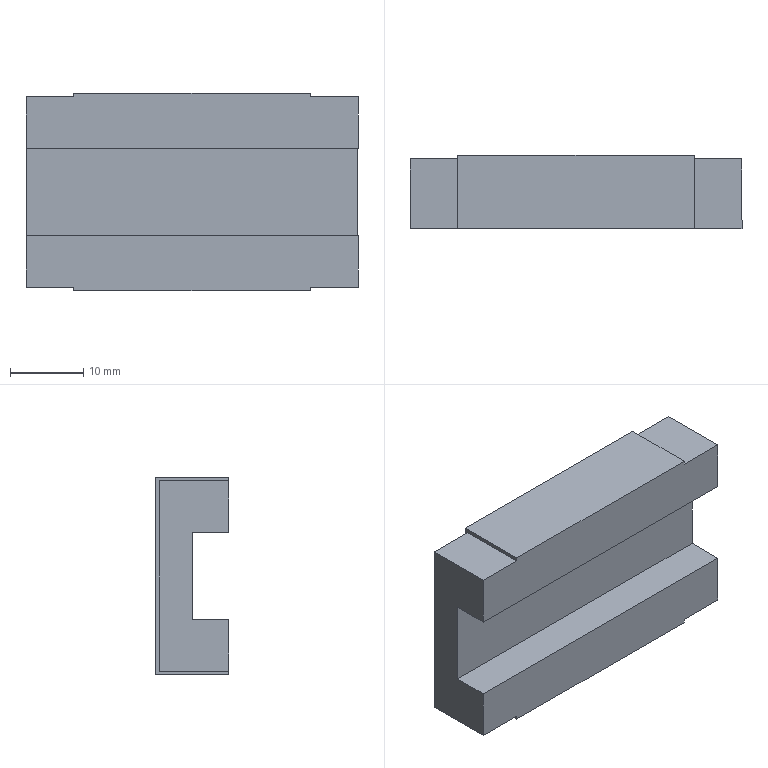Component | SolidWorks | MGN12H1R145Z0C-1_MGN12H-1 | 1 solid | 30 faces | box 45.4 x 10 x 27 mm | volume 9169 mm3 | plane 22 | cylinder 8 | commonest cylinder face diameters 2.3 x8 | material Plain Carbon Steel
build123d program:
from build123d import *

# Parameters (mm, degrees)
SKETCH1_W               = 27
SKETCH1_H               = 10
EXTRUDE1_DEPTH          = 22.7
SKETCH2_W               = 12
SKETCH2_H               = 5
CUT_EXTRUDE1_DEPTH      = 49.409
SKETCH3_W               = 27
SKETCH3_H               = 6.5
CUT_EXTRUDE2_DEPTH      = 0.5
SKETCH4_W               = 0.5
SKETCH4_H               = 6.5
CUT_EXTRUDE3_DEPTH      = 29.068
MIRROR2_COPY_1_SKETCH_W = 0.5
MIRROR2_COPY_1_SKETCH_H = 6.5
MIRROR2_COPY_1_DEPTH    = 29.068
SKETCH5_R               = 1.15
CUT_EXTRUDE4_DEPTH      = 4
LPATTERN1_COUNT         = 2
LPATTERN1_PITCH         = 20
LPATTERN1_COUNT_DIR2    = 2
LPATTERN1_PITCH_DIR2    = 20


with BuildPart() as part:
    # Sketch1 → Extrude1 (new, symmetric)
    with BuildSketch(Plane.XY):
        with Locations((0, 5)):
            Rectangle(SKETCH1_W, SKETCH1_H)
    extrude(amount=EXTRUDE1_DEPTH, both=True)

    # Sketch2 → Cut-Extrude1 (cut, through all)
    with BuildSketch(Plane.XY.offset(22.7)):
        with Locations((0, 2.5)):
            Rectangle(SKETCH2_W, SKETCH2_H)
    extrude(amount=-CUT_EXTRUDE1_DEPTH, mode=Mode.SUBTRACT)

    # Sketch3 → Cut-Extrude2 (cut)
    with BuildSketch(Plane(origin=(0, 10, 0), x_dir=(-1, 0, 0), z_dir=(0, 1, 0))):
        with Locations((0, 19.45)):
            Rectangle(SKETCH3_W, SKETCH3_H)
    cut_extrude2 = extrude(amount=-CUT_EXTRUDE2_DEPTH, mode=Mode.SUBTRACT)

    # Sketch4 → Cut-Extrude3 (cut, through all)
    with BuildSketch(Plane(origin=(0, 9.5, 0), x_dir=(-1, 0, 0), z_dir=(0, 1, 0))):
        with Locations((13.25, 19.45)):
            Rectangle(SKETCH4_W, SKETCH4_H)
    cut_extrude3 = extrude(amount=-CUT_EXTRUDE3_DEPTH, mode=Mode.SUBTRACT)

    # Mirror1: Cut-Extrude3 across plane
    add(cut_extrude3.mirror(Plane(origin=(0, 0, 0), x_dir=(0, 0, 1), z_dir=(1, 0, 0))), mode=Mode.SUBTRACT)

    # Mirror2: Cut-Extrude2, Cut-Extrude3 across plane
    add(cut_extrude2.mirror(Plane.XY), mode=Mode.SUBTRACT)
    add(cut_extrude3.mirror(Plane.XY), mode=Mode.SUBTRACT)

    # Mirror2 copy 1 sketch → Mirror2 copy 1 (cut, through all)
    with BuildSketch(Plane(origin=(0, 9.5, 0), x_dir=(1, 0, 0), z_dir=(0, 1, 0))):
        with Locations((13.25, 19.45)):
            Rectangle(MIRROR2_COPY_1_SKETCH_W, MIRROR2_COPY_1_SKETCH_H)
    extrude(amount=-MIRROR2_COPY_1_DEPTH, mode=Mode.SUBTRACT)

    # Sketch5 → Cut-Extrude4 (cut)
    with BuildSketch(Plane(origin=(0, 10, 0), x_dir=(-1, 0, 0), z_dir=(0, 1, 0))):
        with Locations(Location((-10, 10, 0), (0, 0, 90))):
            Circle(SKETCH5_R)
    cut_extrude4 = extrude(amount=-CUT_EXTRUDE4_DEPTH, mode=Mode.SUBTRACT)

    # LPattern1: Cut-Extrude4 2 × 2
    with Locations(*[(-i * LPATTERN1_PITCH, 0, -j * LPATTERN1_PITCH_DIR2) for i in range(LPATTERN1_COUNT) for j in range(LPATTERN1_COUNT_DIR2) if (i, j) != (0, 0)]):
        add(cut_extrude4, mode=Mode.SUBTRACT)


solid = part.part

# Placed as in the assembly
solid = solid.moved(Location((104.77, 11.768, 38.329), (0, 90, 0)))
STEP:
#1=COLOUR_RGB('',0.7922,0.8196,0.9333);
#2=FILL_AREA_STYLE_COLOUR('',#1);
#3=FILL_AREA_STYLE('',(#2));
#4=SURFACE_STYLE_FILL_AREA(#3);
#5=SURFACE_SIDE_STYLE('',(#4));
#6=SURFACE_STYLE_USAGE(.BOTH.,#5);
#7=PRESENTATION_STYLE_ASSIGNMENT((#6));
#8=CARTESIAN_POINT('',(4.564,0.6995,1.115));
#9=VERTEX_POINT('',#8);
#10=CARTESIAN_POINT('',(4.473,0.6995,1.115));
#11=VERTEX_POINT('',#10);
#12=CARTESIAN_POINT('',(4.519,0.6995,1.115));
#13=DIRECTION('',(-0.,1.,-0.));
#14=DIRECTION('',(-1.,0.,0.));
#15=AXIS2_PLACEMENT_3D('',#12,#13,#14);
#16=CIRCLE('',#15,0.04528);
#17=EDGE_CURVE('',#9,#11,#16,.T.);
#18=ORIENTED_EDGE('',*,*,#17,.F.);
#19=CARTESIAN_POINT('',(4.564,0.857,1.115));
#20=VERTEX_POINT('',#19);
#21=CARTESIAN_POINT('',(4.564,0.6995,1.115));
#22=DIRECTION('',(-0.,1.,-0.));
#23=VECTOR('',#22,39.37);
#24=LINE('',#21,#23);
#25=EDGE_CURVE('',#9,#20,#24,.T.);
#26=ORIENTED_EDGE('',*,*,#25,.T.);
#27=CARTESIAN_POINT('',(4.473,0.857,1.115));
#28=VERTEX_POINT('',#27);
#29=CARTESIAN_POINT('',(4.519,0.857,1.115));
#30=DIRECTION('',(-0.,1.,-0.));
#31=DIRECTION('',(-1.,0.,0.));
#32=AXIS2_PLACEMENT_3D('',#29,#30,#31);
#33=CIRCLE('',#32,0.04528);
#34=EDGE_CURVE('',#20,#28,#33,.T.);
#35=ORIENTED_EDGE('',*,*,#34,.T.);
#36=CARTESIAN_POINT('',(4.473,0.6995,1.115));
#37=DIRECTION('',(-0.,1.,-0.));
#38=VECTOR('',#37,39.37);
#39=LINE('',#36,#38);
#40=EDGE_CURVE('',#11,#28,#39,.T.);
#41=ORIENTED_EDGE('',*,*,#40,.F.);
#42=EDGE_LOOP('',(#18,#26,#35,#41));
#43=FACE_OUTER_BOUND('',#42,.T.);
#44=CARTESIAN_POINT('',(4.519,0.6995,1.115));
#45=DIRECTION('',(-0.,1.,-0.));
#46=DIRECTION('',(-1.,0.,0.));
#47=AXIS2_PLACEMENT_3D('',#44,#45,#46);
#48=CYLINDRICAL_SURFACE('',#47,0.04528);
#49=ADVANCED_FACE('',(#43),#48,.F.);
#50=CARTESIAN_POINT('',(4.564,0.6995,1.903));
#51=VERTEX_POINT('',#50);
#52=CARTESIAN_POINT('',(4.473,0.6995,1.903));
#53=VERTEX_POINT('',#52);
#54=CARTESIAN_POINT('',(4.519,0.6995,1.903));
#55=DIRECTION('',(-0.,1.,-0.));
#56=DIRECTION('',(-1.,0.,0.));
#57=AXIS2_PLACEMENT_3D('',#54,#55,#56);
#58=CIRCLE('',#57,0.04528);
#59=EDGE_CURVE('',#51,#53,#58,.T.);
#60=ORIENTED_EDGE('',*,*,#59,.F.);
#61=CARTESIAN_POINT('',(4.564,0.857,1.903));
#62=VERTEX_POINT('',#61);
#63=CARTESIAN_POINT('',(4.564,0.6995,1.903));
#64=DIRECTION('',(-0.,1.,-0.));
#65=VECTOR('',#64,39.37);
#66=LINE('',#63,#65);
#67=EDGE_CURVE('',#51,#62,#66,.T.);
#68=ORIENTED_EDGE('',*,*,#67,.T.);
#69=CARTESIAN_POINT('',(4.473,0.857,1.903));
#70=VERTEX_POINT('',#69);
#71=CARTESIAN_POINT('',(4.519,0.857,1.903));
#72=DIRECTION('',(-0.,1.,-0.));
#73=DIRECTION('',(-1.,0.,0.));
#74=AXIS2_PLACEMENT_3D('',#71,#72,#73);
#75=CIRCLE('',#74,0.04528);
#76=EDGE_CURVE('',#62,#70,#75,.T.);
#77=ORIENTED_EDGE('',*,*,#76,.T.);
#78=CARTESIAN_POINT('',(4.473,0.6995,1.903));
#79=DIRECTION('',(-0.,1.,-0.));
#80=VECTOR('',#79,39.37);
#81=LINE('',#78,#80);
#82=EDGE_CURVE('',#53,#70,#81,.T.);
#83=ORIENTED_EDGE('',*,*,#82,.F.);
#84=EDGE_LOOP('',(#60,#68,#77,#83));
#85=FACE_OUTER_BOUND('',#84,.T.);
#86=CARTESIAN_POINT('',(4.519,0.6995,1.903));
#87=DIRECTION('',(-0.,1.,-0.));
#88=DIRECTION('',(-1.,0.,0.));
#89=AXIS2_PLACEMENT_3D('',#86,#87,#88);
#90=CYLINDRICAL_SURFACE('',#89,0.04528);
#91=ADVANCED_FACE('',(#85),#90,.F.);
#92=CARTESIAN_POINT('',(3.776,0.6995,1.115));
#93=VERTEX_POINT('',#92);
#94=CARTESIAN_POINT('',(3.686,0.6995,1.115));
#95=VERTEX_POINT('',#94);
#96=CARTESIAN_POINT('',(3.731,0.6995,1.115));
#97=DIRECTION('',(-0.,1.,-0.));
#98=DIRECTION('',(-1.,0.,0.));
#99=AXIS2_PLACEMENT_3D('',#96,#97,#98);
#100=CIRCLE('',#99,0.04528);
#101=EDGE_CURVE('',#93,#95,#100,.T.);
#102=ORIENTED_EDGE('',*,*,#101,.F.);
#103=CARTESIAN_POINT('',(3.776,0.857,1.115));
#104=VERTEX_POINT('',#103);
#105=CARTESIAN_POINT('',(3.776,0.6995,1.115));
#106=DIRECTION('',(-0.,1.,-0.));
#107=VECTOR('',#106,39.37);
#108=LINE('',#105,#107);
#109=EDGE_CURVE('',#93,#104,#108,.T.);
#110=ORIENTED_EDGE('',*,*,#109,.T.);
#111=CARTESIAN_POINT('',(3.686,0.857,1.115));
#112=VERTEX_POINT('',#111);
#113=CARTESIAN_POINT('',(3.731,0.857,1.115));
#114=DIRECTION('',(-0.,1.,-0.));
#115=DIRECTION('',(-1.,0.,0.));
#116=AXIS2_PLACEMENT_3D('',#113,#114,#115);
#117=CIRCLE('',#116,0.04528);
#118=EDGE_CURVE('',#104,#112,#117,.T.);
#119=ORIENTED_EDGE('',*,*,#118,.T.);
#120=CARTESIAN_POINT('',(3.686,0.6995,1.115));
#121=DIRECTION('',(-0.,1.,-0.));
#122=VECTOR('',#121,39.37);
#123=LINE('',#120,#122);
#124=EDGE_CURVE('',#95,#112,#123,.T.);
#125=ORIENTED_EDGE('',*,*,#124,.F.);
#126=EDGE_LOOP('',(#102,#110,#119,#125));
#127=FACE_OUTER_BOUND('',#126,.T.);
#128=CARTESIAN_POINT('',(3.731,0.6995,1.115));
#129=DIRECTION('',(-0.,1.,-0.));
#130=DIRECTION('',(-1.,0.,0.));
#131=AXIS2_PLACEMENT_3D('',#128,#129,#130);
#132=CYLINDRICAL_SURFACE('',#131,0.04528);
#133=ADVANCED_FACE('',(#127),#132,.F.);
#134=CARTESIAN_POINT('',(3.776,0.6995,1.903));
#135=VERTEX_POINT('',#134);
#136=CARTESIAN_POINT('',(3.686,0.6995,1.903));
#137=VERTEX_POINT('',#136);
#138=CARTESIAN_POINT('',(3.731,0.6995,1.903));
#139=DIRECTION('',(-0.,1.,-0.));
#140=DIRECTION('',(-1.,0.,0.));
#141=AXIS2_PLACEMENT_3D('',#138,#139,#140);
#142=CIRCLE('',#141,0.04528);
#143=EDGE_CURVE('',#135,#137,#142,.T.);
#144=ORIENTED_EDGE('',*,*,#143,.F.);
#145=CARTESIAN_POINT('',(3.776,0.857,1.903));
#146=VERTEX_POINT('',#145);
#147=CARTESIAN_POINT('',(3.776,0.6995,1.903));
#148=DIRECTION('',(-0.,1.,-0.));
#149=VECTOR('',#148,39.37);
#150=LINE('',#147,#149);
#151=EDGE_CURVE('',#135,#146,#150,.T.);
#152=ORIENTED_EDGE('',*,*,#151,.T.);
#153=CARTESIAN_POINT('',(3.686,0.857,1.903));
#154=VERTEX_POINT('',#153);
#155=CARTESIAN_POINT('',(3.731,0.857,1.903));
#156=DIRECTION('',(-0.,1.,-0.));
#157=DIRECTION('',(-1.,0.,0.));
#158=AXIS2_PLACEMENT_3D('',#155,#156,#157);
#159=CIRCLE('',#158,0.04528);
#160=EDGE_CURVE('',#146,#154,#159,.T.);
#161=ORIENTED_EDGE('',*,*,#160,.T.);
#162=CARTESIAN_POINT('',(3.686,0.6995,1.903));
#163=DIRECTION('',(-0.,1.,-0.));
#164=VECTOR('',#163,39.37);
#165=LINE('',#162,#164);
#166=EDGE_CURVE('',#137,#154,#165,.T.);
#167=ORIENTED_EDGE('',*,*,#166,.F.);
#168=EDGE_LOOP('',(#144,#152,#161,#167));
#169=FACE_OUTER_BOUND('',#168,.T.);
#170=CARTESIAN_POINT('',(3.731,0.6995,1.903));
#171=DIRECTION('',(-0.,1.,-0.));
#172=DIRECTION('',(-1.,0.,0.));
#173=AXIS2_PLACEMENT_3D('',#170,#171,#172);
#174=CYLINDRICAL_SURFACE('',#173,0.04528);
#175=ADVANCED_FACE('',(#169),#174,.F.);
#176=CARTESIAN_POINT('',(4.763,0.4633,0.9775));
#177=VERTEX_POINT('',#176);
#178=CARTESIAN_POINT('',(4.763,0.857,0.9775));
#179=VERTEX_POINT('',#178);
#180=CARTESIAN_POINT('',(4.763,0.8373,0.9775));
#181=DIRECTION('',(-0.,1.,-0.));
#182=VECTOR('',#181,39.37);
#183=LINE('',#180,#182);
#184=EDGE_CURVE('',#177,#179,#183,.T.);
#185=ORIENTED_EDGE('',*,*,#184,.F.);
#186=CARTESIAN_POINT('',(3.487,0.4633,0.9775));
#187=VERTEX_POINT('',#186);
#188=CARTESIAN_POINT('',(3.231,0.4633,0.9775));
#189=DIRECTION('',(1.,0.,-0.));
#190=VECTOR('',#189,39.37);
#191=LINE('',#188,#190);
#192=EDGE_CURVE('',#187,#177,#191,.T.);
#193=ORIENTED_EDGE('',*,*,#192,.F.);
#194=CARTESIAN_POINT('',(3.487,0.857,0.9775));
#195=VERTEX_POINT('',#194);
#196=CARTESIAN_POINT('',(3.487,0.8373,0.9775));
#197=DIRECTION('',(-0.,1.,-0.));
#198=VECTOR('',#197,39.37);
#199=LINE('',#196,#198);
#200=EDGE_CURVE('',#187,#195,#199,.T.);
#201=ORIENTED_EDGE('',*,*,#200,.T.);
#202=CARTESIAN_POINT('',(3.231,0.857,0.9775));
#203=DIRECTION('',(1.,0.,-0.));
#204=VECTOR('',#203,39.37);
#205=LINE('',#202,#204);
#206=EDGE_CURVE('',#195,#179,#205,.T.);
#207=ORIENTED_EDGE('',*,*,#206,.T.);
#208=EDGE_LOOP('',(#185,#193,#201,#207));
#209=FACE_OUTER_BOUND('',#208,.T.);
#210=CARTESIAN_POINT('',(3.231,0.857,0.9775));
#211=DIRECTION('',(0.,0.,1.));
#212=DIRECTION('',(-0.,1.,-0.));
#213=AXIS2_PLACEMENT_3D('',#210,#211,#212);
#214=PLANE('',#213);
#215=ADVANCED_FACE('',(#209),#214,.F.);
#216=CARTESIAN_POINT('',(5.019,0.4633,0.9972));
#217=VERTEX_POINT('',#216);
#218=CARTESIAN_POINT('',(5.019,0.8373,0.9972));
#219=VERTEX_POINT('',#218);
#220=CARTESIAN_POINT('',(5.019,0.4633,0.9972));
#221=DIRECTION('',(-0.,1.,-0.));
#222=VECTOR('',#221,39.37);
#223=LINE('',#220,#222);
#224=EDGE_CURVE('',#217,#219,#223,.T.);
#225=ORIENTED_EDGE('',*,*,#224,.T.);
#226=CARTESIAN_POINT('',(5.019,0.8373,2.021));
#227=VERTEX_POINT('',#226);
#228=CARTESIAN_POINT('',(5.019,0.8373,2.041));
#229=DIRECTION('',(0.,0.,1.));
#230=VECTOR('',#229,39.37);
#231=LINE('',#228,#230);
#232=EDGE_CURVE('',#219,#227,#231,.T.);
#233=ORIENTED_EDGE('',*,*,#232,.T.);
#234=CARTESIAN_POINT('',(5.019,0.4633,2.021));
#235=VERTEX_POINT('',#234);
#236=CARTESIAN_POINT('',(5.019,0.4633,2.021));
#237=DIRECTION('',(-0.,1.,-0.));
#238=VECTOR('',#237,39.37);
#239=LINE('',#236,#238);
#240=EDGE_CURVE('',#235,#227,#239,.T.);
#241=ORIENTED_EDGE('',*,*,#240,.F.);
#242=CARTESIAN_POINT('',(5.019,0.4633,1.745));
#243=VERTEX_POINT('',#242);
#244=CARTESIAN_POINT('',(5.019,0.4633,0.9775));
#245=DIRECTION('',(0.,0.,1.));
#246=VECTOR('',#245,39.37);
#247=LINE('',#244,#246);
#248=EDGE_CURVE('',#243,#235,#247,.T.);
#249=ORIENTED_EDGE('',*,*,#248,.F.);
#250=CARTESIAN_POINT('',(5.019,0.6602,1.745));
#251=VERTEX_POINT('',#250);
#252=CARTESIAN_POINT('',(5.019,0.6602,1.745));
#253=DIRECTION('',(-0.,1.,-0.));
#254=VECTOR('',#253,39.37);
#255=LINE('',#252,#254);
#256=EDGE_CURVE('',#243,#251,#255,.T.);
#257=ORIENTED_EDGE('',*,*,#256,.T.);
#258=CARTESIAN_POINT('',(5.019,0.6602,1.273));
#259=VERTEX_POINT('',#258);
#260=CARTESIAN_POINT('',(5.019,0.6602,1.273));
#261=DIRECTION('',(-0.,-0.,-1.));
#262=VECTOR('',#261,39.37);
#263=LINE('',#260,#262);
#264=EDGE_CURVE('',#251,#259,#263,.T.);
#265=ORIENTED_EDGE('',*,*,#264,.T.);
#266=CARTESIAN_POINT('',(5.019,0.4633,1.273));
#267=VERTEX_POINT('',#266);
#268=CARTESIAN_POINT('',(5.019,0.6602,1.273));
#269=DIRECTION('',(0.,-1.,0.));
#270=VECTOR('',#269,39.37);
#271=LINE('',#268,#270);
#272=EDGE_CURVE('',#259,#267,#271,.T.);
#273=ORIENTED_EDGE('',*,*,#272,.T.);
#274=CARTESIAN_POINT('',(5.019,0.4633,0.9775));
#275=DIRECTION('',(0.,0.,1.));
#276=VECTOR('',#275,39.37);
#277=LINE('',#274,#276);
#278=EDGE_CURVE('',#217,#267,#277,.T.);
#279=ORIENTED_EDGE('',*,*,#278,.F.);
#280=EDGE_LOOP('',(#225,#233,#241,#249,#257,#265,#273,#279));
#281=FACE_OUTER_BOUND('',#280,.T.);
#282=CARTESIAN_POINT('',(5.019,0.4633,0.9775));
#283=DIRECTION('',(-1.,-0.,0.));
#284=DIRECTION('',(0.,0.,1.));
#285=AXIS2_PLACEMENT_3D('',#282,#283,#284);
#286=PLANE('',#285);
#287=ADVANCED_FACE('',(#281),#286,.F.);
#288=CARTESIAN_POINT('',(4.763,0.4633,0.9972));
#289=VERTEX_POINT('',#288);
#290=CARTESIAN_POINT('',(5.019,0.4633,0.9972));
#291=DIRECTION('',(-1.,-0.,0.));
#292=VECTOR('',#291,39.37);
#293=LINE('',#290,#292);
#294=EDGE_CURVE('',#217,#289,#293,.T.);
#295=ORIENTED_EDGE('',*,*,#294,.F.);
#296=ORIENTED_EDGE('',*,*,#278,.T.);
#297=CARTESIAN_POINT('',(3.231,0.4633,1.273));
#298=VERTEX_POINT('',#297);
#299=CARTESIAN_POINT('',(5.019,0.4633,1.273));
#300=DIRECTION('',(-1.,-0.,0.));
#301=VECTOR('',#300,39.37);
#302=LINE('',#299,#301);
#303=EDGE_CURVE('',#267,#298,#302,.T.);
#304=ORIENTED_EDGE('',*,*,#303,.T.);
#305=CARTESIAN_POINT('',(3.231,0.4633,0.9972));
#306=VERTEX_POINT('',#305);
#307=CARTESIAN_POINT('',(3.231,0.4633,0.9775));
#308=DIRECTION('',(0.,0.,1.));
#309=VECTOR('',#308,39.37);
#310=LINE('',#307,#309);
#311=EDGE_CURVE('',#306,#298,#310,.T.);
#312=ORIENTED_EDGE('',*,*,#311,.F.);
#313=CARTESIAN_POINT('',(3.487,0.4633,0.9972));
#314=VERTEX_POINT('',#313);
#315=CARTESIAN_POINT('',(3.231,0.4633,0.9972));
#316=DIRECTION('',(1.,0.,-0.));
#317=VECTOR('',#316,39.37);
#318=LINE('',#315,#317);
#319=EDGE_CURVE('',#306,#314,#318,.T.);
#320=ORIENTED_EDGE('',*,*,#319,.T.);
#321=CARTESIAN_POINT('',(3.487,0.4633,0.9775));
#322=DIRECTION('',(-0.,-0.,-1.));
#323=VECTOR('',#322,39.37);
#324=LINE('',#321,#323);
#325=EDGE_CURVE('',#314,#187,#324,.T.);
#326=ORIENTED_EDGE('',*,*,#325,.T.);
#327=ORIENTED_EDGE('',*,*,#192,.T.);
#328=CARTESIAN_POINT('',(4.763,0.4633,0.9775));
#329=DIRECTION('',(-0.,-0.,-1.));
#330=VECTOR('',#329,39.37);
#331=LINE('',#328,#330);
#332=EDGE_CURVE('',#289,#177,#331,.T.);
#333=ORIENTED_EDGE('',*,*,#332,.F.);
#334=EDGE_LOOP('',(#295,#296,#304,#312,#320,#326,#327,#333));
#335=FACE_OUTER_BOUND('',#334,.T.);
#336=CARTESIAN_POINT('',(3.231,0.4633,0.9775));
#337=DIRECTION('',(-0.,1.,-0.));
#338=DIRECTION('',(-1.,-0.,0.));
#339=AXIS2_PLACEMENT_3D('',#336,#337,#338);
#340=PLANE('',#339);
#341=ADVANCED_FACE('',(#335),#340,.F.);
#342=ORIENTED_EDGE('',*,*,#232,.F.);
#343=CARTESIAN_POINT('',(4.763,0.8373,0.9972));
#344=VERTEX_POINT('',#343);
#345=CARTESIAN_POINT('',(5.019,0.8373,0.9972));
#346=DIRECTION('',(-1.,-0.,0.));
#347=VECTOR('',#346,39.37);
#348=LINE('',#345,#347);
#349=EDGE_CURVE('',#219,#344,#348,.T.);
#350=ORIENTED_EDGE('',*,*,#349,.T.);
#351=CARTESIAN_POINT('',(4.763,0.8373,2.021));
#352=VERTEX_POINT('',#351);
#353=CARTESIAN_POINT('',(4.763,0.8373,2.041));
#354=DIRECTION('',(-0.,-0.,-1.));
#355=VECTOR('',#354,39.37);
#356=LINE('',#353,#355);
#357=EDGE_CURVE('',#352,#344,#356,.T.);
#358=ORIENTED_EDGE('',*,*,#357,.F.);
#359=CARTESIAN_POINT('',(5.019,0.8373,2.021));
#360=DIRECTION('',(-1.,-0.,0.));
#361=VECTOR('',#360,39.37);
#362=LINE('',#359,#361);
#363=EDGE_CURVE('',#227,#352,#362,.T.);
#364=ORIENTED_EDGE('',*,*,#363,.F.);
#365=EDGE_LOOP('',(#342,#350,#358,#364));
#366=FACE_OUTER_BOUND('',#365,.T.);
#367=CARTESIAN_POINT('',(4.763,0.8373,2.041));
#368=DIRECTION('',(-0.,1.,-0.));
#369=DIRECTION('',(1.,0.,-0.));
#370=AXIS2_PLACEMENT_3D('',#367,#368,#369);
#371=PLANE('',#370);
#372=ADVANCED_FACE('',(#366),#371,.T.);
#373=CARTESIAN_POINT('',(3.487,0.4633,2.041));
#374=VERTEX_POINT('',#373);
#375=CARTESIAN_POINT('',(4.763,0.4633,2.041));
#376=VERTEX_POINT('',#375);
#377=CARTESIAN_POINT('',(3.231,0.4633,2.041));
#378=DIRECTION('',(1.,0.,-0.));
#379=VECTOR('',#378,39.37);
#380=LINE('',#377,#379);
#381=EDGE_CURVE('',#374,#376,#380,.T.);
#382=ORIENTED_EDGE('',*,*,#381,.T.);
#383=CARTESIAN_POINT('',(4.763,0.857,2.041));
#384=VERTEX_POINT('',#383);
#385=CARTESIAN_POINT('',(4.763,0.8373,2.041));
#386=DIRECTION('',(-0.,1.,-0.));
#387=VECTOR('',#386,39.37);
#388=LINE('',#385,#387);
#389=EDGE_CURVE('',#376,#384,#388,.T.);
#390=ORIENTED_EDGE('',*,*,#389,.T.);
#391=CARTESIAN_POINT('',(3.487,0.857,2.041));
#392=VERTEX_POINT('',#391);
#393=CARTESIAN_POINT('',(3.231,0.857,2.041));
#394=DIRECTION('',(1.,0.,-0.));
#395=VECTOR('',#394,39.37);
#396=LINE('',#393,#395);
#397=EDGE_CURVE('',#392,#384,#396,.T.);
#398=ORIENTED_EDGE('',*,*,#397,.F.);
#399=CARTESIAN_POINT('',(3.487,0.8373,2.041));
#400=DIRECTION('',(-0.,1.,-0.));
#401=VECTOR('',#400,39.37);
#402=LINE('',#399,#401);
#403=EDGE_CURVE('',#374,#392,#402,.T.);
#404=ORIENTED_EDGE('',*,*,#403,.F.);
#405=EDGE_LOOP('',(#382,#390,#398,#404));
#406=FACE_OUTER_BOUND('',#405,.T.);
#407=CARTESIAN_POINT('',(3.231,0.857,2.041));
#408=DIRECTION('',(-0.,-0.,-1.));
#409=DIRECTION('',(0.,-1.,0.));
#410=AXIS2_PLACEMENT_3D('',#407,#408,#409);
#411=PLANE('',#410);
#412=ADVANCED_FACE('',(#406),#411,.F.);
#413=CARTESIAN_POINT('',(3.731,0.857,1.115));
#414=DIRECTION('',(-0.,1.,-0.));
#415=DIRECTION('',(-1.,0.,0.));
#416=AXIS2_PLACEMENT_3D('',#413,#414,#415);
#417=CIRCLE('',#416,0.04528);
#418=EDGE_CURVE('',#112,#104,#417,.T.);
#419=ORIENTED_EDGE('',*,*,#418,.F.);
#420=ORIENTED_EDGE('',*,*,#118,.F.);
#421=EDGE_LOOP('',(#419,#420));
#422=FACE_BOUND('',#421,.T.);
#423=CARTESIAN_POINT('',(3.731,0.857,1.903));
#424=DIRECTION('',(-0.,1.,-0.));
#425=DIRECTION('',(-1.,0.,0.));
#426=AXIS2_PLACEMENT_3D('',#423,#424,#425);
#427=CIRCLE('',#426,0.04528);
#428=EDGE_CURVE('',#154,#146,#427,.T.);
#429=ORIENTED_EDGE('',*,*,#428,.F.);
#430=ORIENTED_EDGE('',*,*,#160,.F.);
#431=EDGE_LOOP('',(#429,#430));
#432=FACE_BOUND('',#431,.T.);
#433=CARTESIAN_POINT('',(4.763,0.857,2.041));
#434=DIRECTION('',(-0.,-0.,-1.));
#435=VECTOR('',#434,39.37);
#436=LINE('',#433,#435);
#437=EDGE_CURVE('',#384,#179,#436,.T.);
#438=ORIENTED_EDGE('',*,*,#437,.T.);
#439=ORIENTED_EDGE('',*,*,#206,.F.);
#440=CARTESIAN_POINT('',(3.487,0.857,2.041));
#441=DIRECTION('',(-0.,-0.,-1.));
#442=VECTOR('',#441,39.37);
#443=LINE('',#440,#442);
#444=EDGE_CURVE('',#392,#195,#443,.T.);
#445=ORIENTED_EDGE('',*,*,#444,.F.);
#446=ORIENTED_EDGE('',*,*,#397,.T.);
#447=EDGE_LOOP('',(#438,#439,#445,#446));
#448=FACE_OUTER_BOUND('',#447,.T.);
#449=CARTESIAN_POINT('',(4.519,0.857,1.903));
#450=DIRECTION('',(-0.,1.,-0.));
#451=DIRECTION('',(-1.,0.,0.));
#452=AXIS2_PLACEMENT_3D('',#449,#450,#451);
#453=CIRCLE('',#452,0.04528);
#454=EDGE_CURVE('',#70,#62,#453,.T.);
#455=ORIENTED_EDGE('',*,*,#454,.F.);
#456=ORIENTED_EDGE('',*,*,#76,.F.);
#457=EDGE_LOOP('',(#455,#456));
#458=FACE_BOUND('',#457,.T.);
#459=CARTESIAN_POINT('',(4.519,0.857,1.115));
#460=DIRECTION('',(-0.,1.,-0.));
#461=DIRECTION('',(-1.,0.,0.));
#462=AXIS2_PLACEMENT_3D('',#459,#460,#461);
#463=CIRCLE('',#462,0.04528);
#464=EDGE_CURVE('',#28,#20,#463,.T.);
#465=ORIENTED_EDGE('',*,*,#464,.F.);
#466=ORIENTED_EDGE('',*,*,#34,.F.);
#467=EDGE_LOOP('',(#465,#466));
#468=FACE_BOUND('',#467,.T.);
#469=CARTESIAN_POINT('',(3.231,0.857,0.9775));
#470=DIRECTION('',(0.,-1.,0.));
#471=DIRECTION('',(1.,0.,-0.));
#472=AXIS2_PLACEMENT_3D('',#469,#470,#471);
#473=PLANE('',#472);
#474=ADVANCED_FACE('',(#422,#432,#448,#458,#468),#473,.F.);
#475=CARTESIAN_POINT('',(3.231,0.4633,1.745));
#476=VERTEX_POINT('',#475);
#477=CARTESIAN_POINT('',(3.231,0.4633,2.021));
#478=VERTEX_POINT('',#477);
#479=CARTESIAN_POINT('',(3.231,0.4633,0.9775));
#480=DIRECTION('',(0.,0.,1.));
#481=VECTOR('',#480,39.37);
#482=LINE('',#479,#481);
#483=EDGE_CURVE('',#476,#478,#482,.T.);
#484=ORIENTED_EDGE('',*,*,#483,.T.);
#485=CARTESIAN_POINT('',(3.231,0.8373,2.021));
#486=VERTEX_POINT('',#485);
#487=CARTESIAN_POINT('',(3.231,0.4633,2.021));
#488=DIRECTION('',(-0.,1.,-0.));
#489=VECTOR('',#488,39.37);
#490=LINE('',#487,#489);
#491=EDGE_CURVE('',#478,#486,#490,.T.);
#492=ORIENTED_EDGE('',*,*,#491,.T.);
#493=CARTESIAN_POINT('',(3.231,0.8373,0.9972));
#494=VERTEX_POINT('',#493);
#495=CARTESIAN_POINT('',(3.231,0.8373,2.041));
#496=DIRECTION('',(0.,0.,1.));
#497=VECTOR('',#496,39.37);
#498=LINE('',#495,#497);
#499=EDGE_CURVE('',#494,#486,#498,.T.);
#500=ORIENTED_EDGE('',*,*,#499,.F.);
#501=CARTESIAN_POINT('',(3.231,0.4633,0.9972));
#502=DIRECTION('',(-0.,1.,-0.));
#503=VECTOR('',#502,39.37);
#504=LINE('',#501,#503);
#505=EDGE_CURVE('',#306,#494,#504,.T.);
#506=ORIENTED_EDGE('',*,*,#505,.F.);
#507=ORIENTED_EDGE('',*,*,#311,.T.);
#508=CARTESIAN_POINT('',(3.231,0.6602,1.273));
#509=VERTEX_POINT('',#508);
#510=CARTESIAN_POINT('',(3.231,0.6602,1.273));
#511=DIRECTION('',(0.,-1.,0.));
#512=VECTOR('',#511,39.37);
#513=LINE('',#510,#512);
#514=EDGE_CURVE('',#509,#298,#513,.T.);
#515=ORIENTED_EDGE('',*,*,#514,.F.);
#516=CARTESIAN_POINT('',(3.231,0.6602,1.745));
#517=VERTEX_POINT('',#516);
#518=CARTESIAN_POINT('',(3.231,0.6602,1.273));
#519=DIRECTION('',(-0.,-0.,-1.));
#520=VECTOR('',#519,39.37);
#521=LINE('',#518,#520);
#522=EDGE_CURVE('',#517,#509,#521,.T.);
#523=ORIENTED_EDGE('',*,*,#522,.F.);
#524=CARTESIAN_POINT('',(3.231,0.6602,1.745));
#525=DIRECTION('',(-0.,1.,-0.));
#526=VECTOR('',#525,39.37);
#527=LINE('',#524,#526);
#528=EDGE_CURVE('',#476,#517,#527,.T.);
#529=ORIENTED_EDGE('',*,*,#528,.F.);
#530=EDGE_LOOP('',(#484,#492,#500,#506,#507,#515,#523,#529));
#531=FACE_OUTER_BOUND('',#530,.T.);
#532=CARTESIAN_POINT('',(3.231,0.4633,0.9775));
#533=DIRECTION('',(-1.,-0.,0.));
#534=DIRECTION('',(0.,0.,1.));
#535=AXIS2_PLACEMENT_3D('',#532,#533,#534);
#536=PLANE('',#535);
#537=ADVANCED_FACE('',(#531),#536,.T.);
#538=CARTESIAN_POINT('',(4.763,0.4633,2.021));
#539=VERTEX_POINT('',#538);
#540=CARTESIAN_POINT('',(5.019,0.4633,2.021));
#541=DIRECTION('',(-1.,-0.,0.));
#542=VECTOR('',#541,39.37);
#543=LINE('',#540,#542);
#544=EDGE_CURVE('',#235,#539,#543,.T.);
#545=ORIENTED_EDGE('',*,*,#544,.T.);
#546=CARTESIAN_POINT('',(4.763,0.4633,2.041));
#547=DIRECTION('',(0.,0.,1.));
#548=VECTOR('',#547,39.37);
#549=LINE('',#546,#548);
#550=EDGE_CURVE('',#539,#376,#549,.T.);
#551=ORIENTED_EDGE('',*,*,#550,.T.);
#552=ORIENTED_EDGE('',*,*,#381,.F.);
#553=CARTESIAN_POINT('',(3.487,0.4633,2.021));
#554=VERTEX_POINT('',#553);
#555=CARTESIAN_POINT('',(3.487,0.4633,2.041));
#556=DIRECTION('',(0.,0.,1.));
#557=VECTOR('',#556,39.37);
#558=LINE('',#555,#557);
#559=EDGE_CURVE('',#554,#374,#558,.T.);
#560=ORIENTED_EDGE('',*,*,#559,.F.);
#561=CARTESIAN_POINT('',(3.231,0.4633,2.021));
#562=DIRECTION('',(1.,0.,-0.));
#563=VECTOR('',#562,39.37);
#564=LINE('',#561,#563);
#565=EDGE_CURVE('',#478,#554,#564,.T.);
#566=ORIENTED_EDGE('',*,*,#565,.F.);
#567=ORIENTED_EDGE('',*,*,#483,.F.);
#568=CARTESIAN_POINT('',(5.019,0.4633,1.745));
#569=DIRECTION('',(-1.,-0.,0.));
#570=VECTOR('',#569,39.37);
#571=LINE('',#568,#570);
#572=EDGE_CURVE('',#243,#476,#571,.T.);
#573=ORIENTED_EDGE('',*,*,#572,.F.);
#574=ORIENTED_EDGE('',*,*,#248,.T.);
#575=EDGE_LOOP('',(#545,#551,#552,#560,#566,#567,#573,#574));
#576=FACE_OUTER_BOUND('',#575,.T.);
#577=CARTESIAN_POINT('',(3.231,0.4633,0.9775));
#578=DIRECTION('',(-0.,1.,-0.));
#579=DIRECTION('',(-1.,-0.,0.));
#580=AXIS2_PLACEMENT_3D('',#577,#578,#579);
#581=PLANE('',#580);
#582=ADVANCED_FACE('',(#576),#581,.F.);
#583=ORIENTED_EDGE('',*,*,#499,.T.);
#584=CARTESIAN_POINT('',(3.487,0.8373,2.021));
#585=VERTEX_POINT('',#584);
#586=CARTESIAN_POINT('',(3.231,0.8373,2.021));
#587=DIRECTION('',(1.,0.,-0.));
#588=VECTOR('',#587,39.37);
#589=LINE('',#586,#588);
#590=EDGE_CURVE('',#486,#585,#589,.T.);
#591=ORIENTED_EDGE('',*,*,#590,.T.);
#592=CARTESIAN_POINT('',(3.487,0.8373,0.9972));
#593=VERTEX_POINT('',#592);
#594=CARTESIAN_POINT('',(3.487,0.8373,2.041));
#595=DIRECTION('',(-0.,-0.,-1.));
#596=VECTOR('',#595,39.37);
#597=LINE('',#594,#596);
#598=EDGE_CURVE('',#585,#593,#597,.T.);
#599=ORIENTED_EDGE('',*,*,#598,.T.);
#600=CARTESIAN_POINT('',(3.231,0.8373,0.9972));
#601=DIRECTION('',(1.,0.,-0.));
#602=VECTOR('',#601,39.37);
#603=LINE('',#600,#602);
#604=EDGE_CURVE('',#494,#593,#603,.T.);
#605=ORIENTED_EDGE('',*,*,#604,.F.);
#606=EDGE_LOOP('',(#583,#591,#599,#605));
#607=FACE_OUTER_BOUND('',#606,.T.);
#608=CARTESIAN_POINT('',(3.487,0.8373,2.041));
#609=DIRECTION('',(-0.,1.,-0.));
#610=DIRECTION('',(-1.,-0.,0.));
#611=AXIS2_PLACEMENT_3D('',#608,#609,#610);
#612=PLANE('',#611);
#613=ADVANCED_FACE('',(#607),#612,.T.);
#614=ORIENTED_EDGE('',*,*,#514,.T.);
#615=ORIENTED_EDGE('',*,*,#303,.F.);
#616=ORIENTED_EDGE('',*,*,#272,.F.);
#617=CARTESIAN_POINT('',(5.019,0.6602,1.273));
#618=DIRECTION('',(-1.,-0.,0.));
#619=VECTOR('',#618,39.37);
#620=LINE('',#617,#619);
#621=EDGE_CURVE('',#259,#509,#620,.T.);
#622=ORIENTED_EDGE('',*,*,#621,.T.);
#623=EDGE_LOOP('',(#614,#615,#616,#622));
#624=FACE_OUTER_BOUND('',#623,.T.);
#625=CARTESIAN_POINT('',(5.019,0.6602,1.273));
#626=DIRECTION('',(-0.,-0.,-1.));
#627=DIRECTION('',(0.,-1.,0.));
#628=AXIS2_PLACEMENT_3D('',#625,#626,#627);
#629=PLANE('',#628);
#630=ADVANCED_FACE('',(#624),#629,.F.);
#631=ORIENTED_EDGE('',*,*,#522,.T.);
#632=ORIENTED_EDGE('',*,*,#621,.F.);
#633=ORIENTED_EDGE('',*,*,#264,.F.);
#634=CARTESIAN_POINT('',(5.019,0.6602,1.745));
#635=DIRECTION('',(-1.,-0.,0.));
#636=VECTOR('',#635,39.37);
#637=LINE('',#634,#636);
#638=EDGE_CURVE('',#251,#517,#637,.T.);
#639=ORIENTED_EDGE('',*,*,#638,.T.);
#640=EDGE_LOOP('',(#631,#632,#633,#639));
#641=FACE_OUTER_BOUND('',#640,.T.);
#642=CARTESIAN_POINT('',(5.019,0.6602,1.273));
#643=DIRECTION('',(-0.,1.,-0.));
#644=DIRECTION('',(-1.,-0.,0.));
#645=AXIS2_PLACEMENT_3D('',#642,#643,#644);
#646=PLANE('',#645);
#647=ADVANCED_FACE('',(#641),#646,.F.);
#648=ORIENTED_EDGE('',*,*,#528,.T.);
#649=ORIENTED_EDGE('',*,*,#638,.F.);
#650=ORIENTED_EDGE('',*,*,#256,.F.);
#651=ORIENTED_EDGE('',*,*,#572,.T.);
#652=EDGE_LOOP('',(#648,#649,#650,#651));
#653=FACE_OUTER_BOUND('',#652,.T.);
#654=CARTESIAN_POINT('',(5.019,0.6602,1.745));
#655=DIRECTION('',(0.,0.,1.));
#656=DIRECTION('',(-0.,1.,-0.));
#657=AXIS2_PLACEMENT_3D('',#654,#655,#656);
#658=PLANE('',#657);
#659=ADVANCED_FACE('',(#653),#658,.F.);
#660=ORIENTED_EDGE('',*,*,#444,.T.);
#661=ORIENTED_EDGE('',*,*,#200,.F.);
#662=ORIENTED_EDGE('',*,*,#325,.F.);
#663=CARTESIAN_POINT('',(3.487,0.4633,0.9972));
#664=DIRECTION('',(-0.,1.,-0.));
#665=VECTOR('',#664,39.37);
#666=LINE('',#663,#665);
#667=EDGE_CURVE('',#314,#593,#666,.T.);
#668=ORIENTED_EDGE('',*,*,#667,.T.);
#669=ORIENTED_EDGE('',*,*,#598,.F.);
#670=CARTESIAN_POINT('',(3.487,0.4633,2.021));
#671=DIRECTION('',(-0.,1.,-0.));
#672=VECTOR('',#671,39.37);
#673=LINE('',#670,#672);
#674=EDGE_CURVE('',#554,#585,#673,.T.);
#675=ORIENTED_EDGE('',*,*,#674,.F.);
#676=ORIENTED_EDGE('',*,*,#559,.T.);
#677=ORIENTED_EDGE('',*,*,#403,.T.);
#678=EDGE_LOOP('',(#660,#661,#662,#668,#669,#675,#676,#677));
#679=FACE_OUTER_BOUND('',#678,.T.);
#680=CARTESIAN_POINT('',(3.487,0.8373,2.041));
#681=DIRECTION('',(1.,0.,-0.));
#682=DIRECTION('',(-0.,-0.,-1.));
#683=AXIS2_PLACEMENT_3D('',#680,#681,#682);
#684=PLANE('',#683);
#685=ADVANCED_FACE('',(#679),#684,.F.);
#686=ORIENTED_EDGE('',*,*,#604,.T.);
#687=ORIENTED_EDGE('',*,*,#667,.F.);
#688=ORIENTED_EDGE('',*,*,#319,.F.);
#689=ORIENTED_EDGE('',*,*,#505,.T.);
#690=EDGE_LOOP('',(#686,#687,#688,#689));
#691=FACE_OUTER_BOUND('',#690,.T.);
#692=CARTESIAN_POINT('',(3.231,0.4633,0.9972));
#693=DIRECTION('',(0.,0.,1.));
#694=DIRECTION('',(1.,0.,-0.));
#695=AXIS2_PLACEMENT_3D('',#692,#693,#694);
#696=PLANE('',#695);
#697=ADVANCED_FACE('',(#691),#696,.F.);
#698=ORIENTED_EDGE('',*,*,#590,.F.);
#699=ORIENTED_EDGE('',*,*,#491,.F.);
#700=ORIENTED_EDGE('',*,*,#565,.T.);
#701=ORIENTED_EDGE('',*,*,#674,.T.);
#702=EDGE_LOOP('',(#698,#699,#700,#701));
#703=FACE_OUTER_BOUND('',#702,.T.);
#704=CARTESIAN_POINT('',(3.231,0.4633,2.021));
#705=DIRECTION('',(0.,0.,1.));
#706=DIRECTION('',(1.,0.,-0.));
#707=AXIS2_PLACEMENT_3D('',#704,#705,#706);
#708=PLANE('',#707);
#709=ADVANCED_FACE('',(#703),#708,.T.);
#710=ORIENTED_EDGE('',*,*,#437,.F.);
#711=ORIENTED_EDGE('',*,*,#389,.F.);
#712=ORIENTED_EDGE('',*,*,#550,.F.);
#713=CARTESIAN_POINT('',(4.763,0.4633,2.021));
#714=DIRECTION('',(-0.,1.,-0.));
#715=VECTOR('',#714,39.37);
#716=LINE('',#713,#715);
#717=EDGE_CURVE('',#539,#352,#716,.T.);
#718=ORIENTED_EDGE('',*,*,#717,.T.);
#719=ORIENTED_EDGE('',*,*,#357,.T.);
#720=CARTESIAN_POINT('',(4.763,0.4633,0.9972));
#721=DIRECTION('',(-0.,1.,-0.));
#722=VECTOR('',#721,39.37);
#723=LINE('',#720,#722);
#724=EDGE_CURVE('',#289,#344,#723,.T.);
#725=ORIENTED_EDGE('',*,*,#724,.F.);
#726=ORIENTED_EDGE('',*,*,#332,.T.);
#727=ORIENTED_EDGE('',*,*,#184,.T.);
#728=EDGE_LOOP('',(#710,#711,#712,#718,#719,#725,#726,#727));
#729=FACE_OUTER_BOUND('',#728,.T.);
#730=CARTESIAN_POINT('',(4.763,0.8373,2.041));
#731=DIRECTION('',(1.,0.,-0.));
#732=DIRECTION('',(-0.,-0.,-1.));
#733=AXIS2_PLACEMENT_3D('',#730,#731,#732);
#734=PLANE('',#733);
#735=ADVANCED_FACE('',(#729),#734,.T.);
#736=ORIENTED_EDGE('',*,*,#363,.T.);
#737=ORIENTED_EDGE('',*,*,#717,.F.);
#738=ORIENTED_EDGE('',*,*,#544,.F.);
#739=ORIENTED_EDGE('',*,*,#240,.T.);
#740=EDGE_LOOP('',(#736,#737,#738,#739));
#741=FACE_OUTER_BOUND('',#740,.T.);
#742=CARTESIAN_POINT('',(5.019,0.4633,2.021));
#743=DIRECTION('',(-0.,-0.,-1.));
#744=DIRECTION('',(-1.,-0.,0.));
#745=AXIS2_PLACEMENT_3D('',#742,#743,#744);
#746=PLANE('',#745);
#747=ADVANCED_FACE('',(#741),#746,.F.);
#748=ORIENTED_EDGE('',*,*,#349,.F.);
#749=ORIENTED_EDGE('',*,*,#224,.F.);
#750=ORIENTED_EDGE('',*,*,#294,.T.);
#751=ORIENTED_EDGE('',*,*,#724,.T.);
#752=EDGE_LOOP('',(#748,#749,#750,#751));
#753=FACE_OUTER_BOUND('',#752,.T.);
#754=CARTESIAN_POINT('',(5.019,0.4633,0.9972));
#755=DIRECTION('',(-0.,-0.,-1.));
#756=DIRECTION('',(-1.,-0.,0.));
#757=AXIS2_PLACEMENT_3D('',#754,#755,#756);
#758=PLANE('',#757);
#759=ADVANCED_FACE('',(#753),#758,.T.);
#760=ORIENTED_EDGE('',*,*,#151,.F.);
#761=CARTESIAN_POINT('',(3.731,0.6995,1.903));
#762=DIRECTION('',(-0.,1.,-0.));
#763=DIRECTION('',(-1.,0.,0.));
#764=AXIS2_PLACEMENT_3D('',#761,#762,#763);
#765=CIRCLE('',#764,0.04528);
#766=EDGE_CURVE('',#137,#135,#765,.T.);
#767=ORIENTED_EDGE('',*,*,#766,.F.);
#768=ORIENTED_EDGE('',*,*,#166,.T.);
#769=ORIENTED_EDGE('',*,*,#428,.T.);
#770=EDGE_LOOP('',(#760,#767,#768,#769));
#771=FACE_OUTER_BOUND('',#770,.T.);
#772=CARTESIAN_POINT('',(3.731,0.6995,1.903));
#773=DIRECTION('',(-0.,1.,-0.));
#774=DIRECTION('',(-1.,0.,0.));
#775=AXIS2_PLACEMENT_3D('',#772,#773,#774);
#776=CYLINDRICAL_SURFACE('',#775,0.04528);
#777=ADVANCED_FACE('',(#771),#776,.F.);
#778=ORIENTED_EDGE('',*,*,#766,.T.);
#779=ORIENTED_EDGE('',*,*,#143,.T.);
#780=EDGE_LOOP('',(#778,#779));
#781=FACE_OUTER_BOUND('',#780,.T.);
#782=CARTESIAN_POINT('',(3.731,0.6995,1.903));
#783=DIRECTION('',(-0.,1.,-0.));
#784=DIRECTION('',(-1.,-0.,0.));
#785=AXIS2_PLACEMENT_3D('',#782,#783,#784);
#786=PLANE('',#785);
#787=ADVANCED_FACE('',(#781),#786,.T.);
#788=ORIENTED_EDGE('',*,*,#109,.F.);
#789=CARTESIAN_POINT('',(3.731,0.6995,1.115));
#790=DIRECTION('',(-0.,1.,-0.));
#791=DIRECTION('',(-1.,0.,0.));
#792=AXIS2_PLACEMENT_3D('',#789,#790,#791);
#793=CIRCLE('',#792,0.04528);
#794=EDGE_CURVE('',#95,#93,#793,.T.);
#795=ORIENTED_EDGE('',*,*,#794,.F.);
#796=ORIENTED_EDGE('',*,*,#124,.T.);
#797=ORIENTED_EDGE('',*,*,#418,.T.);
#798=EDGE_LOOP('',(#788,#795,#796,#797));
#799=FACE_OUTER_BOUND('',#798,.T.);
#800=CARTESIAN_POINT('',(3.731,0.6995,1.115));
#801=DIRECTION('',(-0.,1.,-0.));
#802=DIRECTION('',(-1.,0.,0.));
#803=AXIS2_PLACEMENT_3D('',#800,#801,#802);
#804=CYLINDRICAL_SURFACE('',#803,0.04528);
#805=ADVANCED_FACE('',(#799),#804,.F.);
#806=ORIENTED_EDGE('',*,*,#794,.T.);
#807=ORIENTED_EDGE('',*,*,#101,.T.);
#808=EDGE_LOOP('',(#806,#807));
#809=FACE_OUTER_BOUND('',#808,.T.);
#810=CARTESIAN_POINT('',(3.731,0.6995,1.115));
#811=DIRECTION('',(-0.,1.,-0.));
#812=DIRECTION('',(-1.,-0.,0.));
#813=AXIS2_PLACEMENT_3D('',#810,#811,#812);
#814=PLANE('',#813);
#815=ADVANCED_FACE('',(#809),#814,.T.);
#816=CARTESIAN_POINT('',(4.519,0.6995,1.903));
#817=DIRECTION('',(-0.,1.,-0.));
#818=DIRECTION('',(-1.,0.,0.));
#819=AXIS2_PLACEMENT_3D('',#816,#817,#818);
#820=CIRCLE('',#819,0.04528);
#821=EDGE_CURVE('',#53,#51,#820,.T.);
#822=ORIENTED_EDGE('',*,*,#821,.T.);
#823=ORIENTED_EDGE('',*,*,#59,.T.);
#824=EDGE_LOOP('',(#822,#823));
#825=FACE_OUTER_BOUND('',#824,.T.);
#826=CARTESIAN_POINT('',(4.519,0.6995,1.903));
#827=DIRECTION('',(-0.,1.,-0.));
#828=DIRECTION('',(-1.,-0.,0.));
#829=AXIS2_PLACEMENT_3D('',#826,#827,#828);
#830=PLANE('',#829);
#831=ADVANCED_FACE('',(#825),#830,.T.);
#832=ORIENTED_EDGE('',*,*,#67,.F.);
#833=ORIENTED_EDGE('',*,*,#821,.F.);
#834=ORIENTED_EDGE('',*,*,#82,.T.);
#835=ORIENTED_EDGE('',*,*,#454,.T.);
#836=EDGE_LOOP('',(#832,#833,#834,#835));
#837=FACE_OUTER_BOUND('',#836,.T.);
#838=CARTESIAN_POINT('',(4.519,0.6995,1.903));
#839=DIRECTION('',(-0.,1.,-0.));
#840=DIRECTION('',(-1.,0.,0.));
#841=AXIS2_PLACEMENT_3D('',#838,#839,#840);
#842=CYLINDRICAL_SURFACE('',#841,0.04528);
#843=ADVANCED_FACE('',(#837),#842,.F.);
#844=CARTESIAN_POINT('',(4.519,0.6995,1.115));
#845=DIRECTION('',(-0.,1.,-0.));
#846=DIRECTION('',(-1.,0.,0.));
#847=AXIS2_PLACEMENT_3D('',#844,#845,#846);
#848=CIRCLE('',#847,0.04528);
#849=EDGE_CURVE('',#11,#9,#848,.T.);
#850=ORIENTED_EDGE('',*,*,#849,.T.);
#851=ORIENTED_EDGE('',*,*,#17,.T.);
#852=EDGE_LOOP('',(#850,#851));
#853=FACE_OUTER_BOUND('',#852,.T.);
#854=CARTESIAN_POINT('',(4.519,0.6995,1.115));
#855=DIRECTION('',(-0.,1.,-0.));
#856=DIRECTION('',(-1.,-0.,0.));
#857=AXIS2_PLACEMENT_3D('',#854,#855,#856);
#858=PLANE('',#857);
#859=ADVANCED_FACE('',(#853),#858,.T.);
#860=ORIENTED_EDGE('',*,*,#25,.F.);
#861=ORIENTED_EDGE('',*,*,#849,.F.);
#862=ORIENTED_EDGE('',*,*,#40,.T.);
#863=ORIENTED_EDGE('',*,*,#464,.T.);
#864=EDGE_LOOP('',(#860,#861,#862,#863));
#865=FACE_OUTER_BOUND('',#864,.T.);
#866=CARTESIAN_POINT('',(4.519,0.6995,1.115));
#867=DIRECTION('',(-0.,1.,-0.));
#868=DIRECTION('',(-1.,0.,0.));
#869=AXIS2_PLACEMENT_3D('',#866,#867,#868);
#870=CYLINDRICAL_SURFACE('',#869,0.04528);
#871=ADVANCED_FACE('',(#865),#870,.F.);
#872=CLOSED_SHELL('',(#49,#91,#133,#175,#215,#287,#341,#372,#412,#474,#537,#582,#613,#630,#647,#659,#685,#697,#709,#735,#747,#759,#777,#787,#805,#815,#831,#843,#859,#871));
#873=MANIFOLD_SOLID_BREP('',#872);
#874=STYLED_ITEM('',(#7),#873);
#875=(LENGTH_UNIT()NAMED_UNIT(*)SI_UNIT($,.METRE.));
#876=LENGTH_MEASURE_WITH_UNIT(LENGTH_MEASURE(0.0254),#875);
#877=DIMENSIONAL_EXPONENTS(1.,0.,0.,0.,0.,0.,0.);
#878=(CONVERSION_BASED_UNIT('',#876)LENGTH_UNIT()NAMED_UNIT(#877));
#879=UNCERTAINTY_MEASURE_WITH_UNIT(LENGTH_MEASURE(0.00001),#878,'','');
#880=(NAMED_UNIT(*)PLANE_ANGLE_UNIT()SI_UNIT($,.RADIAN.));
#881=(NAMED_UNIT(*)SI_UNIT($,.STERADIAN.)SOLID_ANGLE_UNIT());
#882=(GEOMETRIC_REPRESENTATION_CONTEXT(3)GLOBAL_UNCERTAINTY_ASSIGNED_CONTEXT((#879))GLOBAL_UNIT_ASSIGNED_CONTEXT((#878,#880,#881))REPRESENTATION_CONTEXT('',''));
#883=MECHANICAL_DESIGN_GEOMETRIC_PRESENTATION_REPRESENTATION('',(#874),#882);
#884=CARTESIAN_POINT('',(0.,0.,0.));
#885=DIRECTION('',(0.,0.,1.));
#886=DIRECTION('',(1.,0.,0.));
#887=AXIS2_PLACEMENT_3D('',#884,#885,#886);
#888=(LENGTH_UNIT()NAMED_UNIT(*)SI_UNIT($,.METRE.));
#889=LENGTH_MEASURE_WITH_UNIT(LENGTH_MEASURE(0.0254),#888);
#890=DIMENSIONAL_EXPONENTS(1.,0.,0.,0.,0.,0.,0.);
#891=(CONVERSION_BASED_UNIT('',#889)LENGTH_UNIT()NAMED_UNIT(#890));
#892=UNCERTAINTY_MEASURE_WITH_UNIT(LENGTH_MEASURE(0.00001),#891,'','');
#893=(NAMED_UNIT(*)PLANE_ANGLE_UNIT()SI_UNIT($,.RADIAN.));
#894=(NAMED_UNIT(*)SI_UNIT($,.STERADIAN.)SOLID_ANGLE_UNIT());
#895=(GEOMETRIC_REPRESENTATION_CONTEXT(3)GLOBAL_UNCERTAINTY_ASSIGNED_CONTEXT((#892))GLOBAL_UNIT_ASSIGNED_CONTEXT((#891,#893,#894))REPRESENTATION_CONTEXT('',''));
#896=ADVANCED_BREP_SHAPE_REPRESENTATION('',(#873,#887),#895);
#897=PRESENTATION_LAYER_ASSIGNMENT('','',(#874));